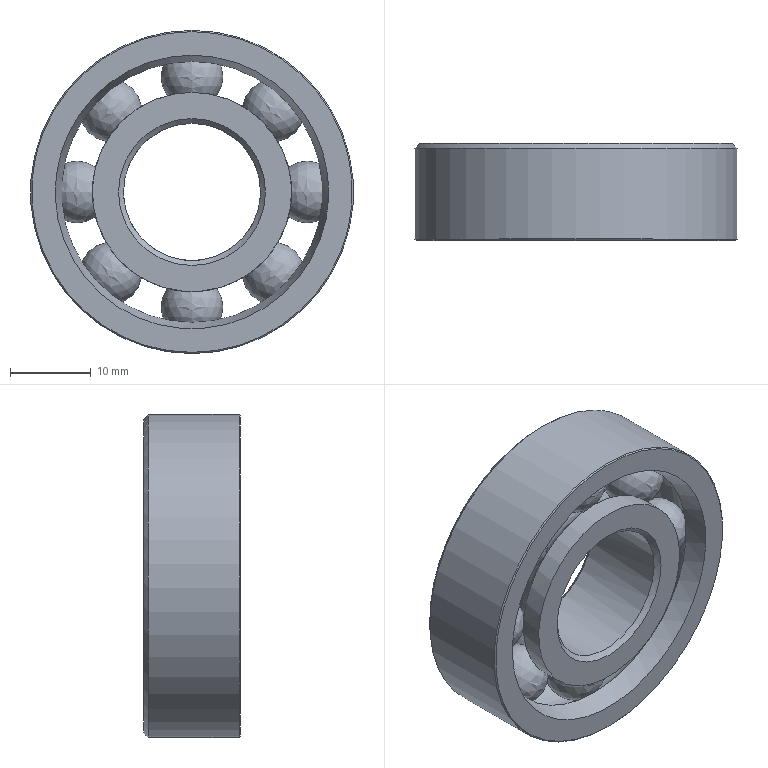Component | NX | BEARING | 10 solids | 24 faces | volume 8359 mm3 | sphere 8 | cylinder 5 | cone 5 | plane 4 | torus 2 | commonest cylinder face diameters 24.667 x2 40 x1 32.333 x1 17 x1